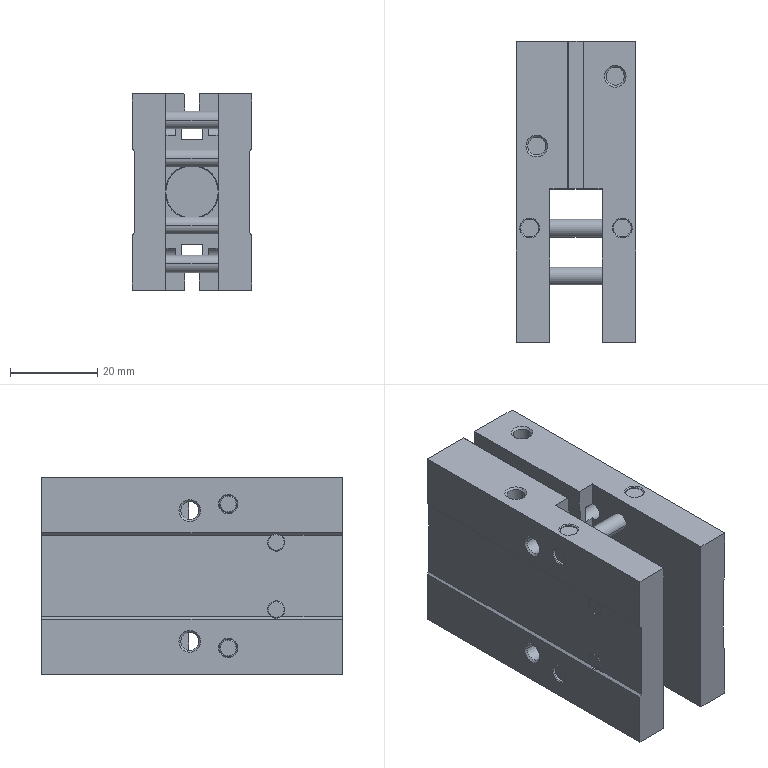Component | SolidWorks | CCDJSHFP20(NC)+(CS1-G-2)-1_CCDJSHFP20_body-1 | 1 solid | 186 faces | box 27.5 x 69 x 45 mm | volume 54359 mm3 | plane 66 | cylinder 64 | cone 56 | commonest cylinder face diameters 4 x32 4.134 x20 2 x4 21 x2 17.4 x2 20 x2 12 x2
build123d program:
from build123d import *

# Parameters (mm, degrees)
BOSS_EXTRUDE1_DEPTH     = 69
CUT_EXTRUDE1_DEPTH      = 22.5
CUT_EXTRUDE1_DEPTH_BACK = 22.5
SKETCH2_W               = 35.2
SKETCH2_H               = 12
LPATTERN1_COUNT         = 2
LPATTERN1_PITCH         = 36.715


with BuildPart() as part:
    # Sketch1 → Boss-Extrude1 (new body)
    with BuildSketch(Plane(origin=(0, 0, 0), x_dir=(0, 0, -1), z_dir=(1, 0, 0))):
        Polygon((-13.75, 9.9), (-13.25, 9.4), (-13.25, -9.4), (-13.75, -9.9), (-13.75, -22.5), (-1.9, -22.5), (-1.7, -22.3), (-1.7, -16.7), (-2.3, -16.7), (-2.3, -12), (2.3, -12), (2.3, -16.7), (1.7, -16.7), (1.7, -22.5), (13.75, -22.5), (13.75, -9.9), (13.25, -9.4), (13.25, 9.4), (13.75, 9.9), (13.75, 22.5), (1.7, 22.5), (1.7, 16.7), (2.3, 16.7), (2.3, 12), (-2.3, 12), (-2.3, 16.7), (-1.7, 16.7), (-1.7, 22.5), (-13.75, 22.5), align=None)
    extrude(amount=BOSS_EXTRUDE1_DEPTH)

    # Sketch2 → Cut-Extrude1 (cut, two sides: drawn at the far end of the back side and taken through both)
    with BuildSketch(Plane(origin=(0, 0, 0), x_dir=(1, 0, 0), z_dir=(0, 1, 0)).offset(-CUT_EXTRUDE1_DEPTH_BACK)):
        with Locations((17.6, 0)):
            Rectangle(SKETCH2_W, SKETCH2_H)
    extrude(amount=CUT_EXTRUDE1_DEPTH + CUT_EXTRUDE1_DEPTH_BACK, mode=Mode.SUBTRACT)

    # Sketch3 → Cut-Revolve1 (revolve, cut)
    with BuildSketch(Plane.XY, mode=Mode.PRIVATE) as cut_revolve1_sk:
        Polygon((35.2, 0), (35.2, 6.2), (35.4, 6), (43.9, 6), (43.9, 10), (61.2, 10), (61.2, 0), align=None)
    revolve(cut_revolve1_sk.sketch.rotate(Axis((61.2, 0, 0), (-1, 0, 0)), 270), axis=Axis((61.2, 0, 0), (-1, 0, 0)), mode=Mode.SUBTRACT)

    # Sketch4 → Cut-Revolve2 (revolve, cut)
    with BuildSketch(Plane.XY, mode=Mode.PRIVATE) as cut_revolve2_sk:
        Polygon((66.6, 0), (66.6, 8.7), (67.8, 8.7), (67.8, 10.5), (68.8, 10.5), (69, 10.7), (69, 0), align=None)
    revolve(cut_revolve2_sk.sketch.rotate(Axis((69, 0, 0), (-1, 0, 0)), 180), axis=Axis((69, 0, 0), (-1, 0, 0)), mode=Mode.SUBTRACT)

    # Sketch5 → Cut-Revolve3 (revolve, cut)
    with BuildSketch(Plane(origin=(35, 0, 0), x_dir=(0, 0, -1), z_dir=(1, 0, 0)), mode=Mode.PRIVATE) as cut_revolve3_sk:
        Polygon((-13.75, 15), (-13.75, 17.5), (-13.317, 17.067), (-3.75, 17.067), (-3.75, 15), align=None)
    revolve(cut_revolve3_sk.sketch.rotate(Axis((35, 15, 3.75), (0, 0, 1)), 270), axis=Axis((35, 15, 3.75), (0, 0, 1)), mode=Mode.SUBTRACT)

    # Sketch6 → Cut-Revolve4 (revolve, cut)
    with BuildSketch(Plane(origin=(35, 0, 0), x_dir=(0, 0, -1), z_dir=(1, 0, 0)), mode=Mode.PRIVATE) as cut_revolve4_sk:
        Polygon((3.75, 15), (3.75, 17.067), (13.317, 17.067), (13.75, 17.5), (13.75, 15), align=None)
    revolve(cut_revolve4_sk.sketch.rotate(Axis((35, 15, -13.75), (0, 0, 1)), 270), axis=Axis((35, 15, -13.75), (0, 0, 1)), mode=Mode.SUBTRACT)

    # Sketch7 → Cut-Revolve5 (revolve, cut)
    with BuildSketch(Plane(origin=(35, 0, 0), x_dir=(0, 0, -1), z_dir=(1, 0, 0)), mode=Mode.PRIVATE) as cut_revolve5_sk:
        Polygon((-13.75, -15), (-13.75, -12.5), (-13.317, -12.933), (-3.75, -12.933), (-3.75, -15), align=None)
    revolve(cut_revolve5_sk.sketch.rotate(Axis((35, -15, 3.75), (0, 0, 1)), 270), axis=Axis((35, -15, 3.75), (0, 0, 1)), mode=Mode.SUBTRACT)

    # Sketch8 → Cut-Revolve6 (revolve, cut)
    with BuildSketch(Plane(origin=(35, 0, 0), x_dir=(0, 0, -1), z_dir=(1, 0, 0)), mode=Mode.PRIVATE) as cut_revolve6_sk:
        Polygon((3.75, -15), (3.75, -12.933), (13.317, -12.933), (13.75, -12.5), (13.75, -15), align=None)
    revolve(cut_revolve6_sk.sketch.rotate(Axis((35, -15, -13.75), (0, 0, 1)), 270), axis=Axis((35, -15, -13.75), (0, 0, 1)), mode=Mode.SUBTRACT)

    # Sketch9 → Cut-Revolve7 (revolve, cut)
    with BuildSketch(Plane.XY.offset(7.5), mode=Mode.PRIVATE) as cut_revolve7_sk:
        Polygon((61.5, 9), (60.5, 9), (60.5, 12), (59.433, 12), (59.433, 22.067), (59, 22.5), (61.5, 22.5), align=None)
    revolve(cut_revolve7_sk.sketch.rotate(Axis((61.5, 22.5, 7.5), (0, -1, 0)), 90), axis=Axis((61.5, 22.5, 7.5), (0, -1, 0)), mode=Mode.SUBTRACT)

    # Sketch10 → Cut-Revolve8 (revolve, cut)
    with BuildSketch(Plane.XY.offset(-7.5), mode=Mode.PRIVATE) as cut_revolve8_sk:
        Polygon((45, 9), (44, 9), (44, 12), (42.933, 12), (42.933, 22.067), (42.5, 22.5), (45, 22.5), align=None)
    revolve(cut_revolve8_sk.sketch.rotate(Axis((45, 22.5, -7.5), (0, -1, 0)), 90), axis=Axis((45, 22.5, -7.5), (0, -1, 0)), mode=Mode.SUBTRACT)

    # Sketch11 → Cut-Revolve9 (revolve, cut)
    with BuildSketch(Plane(origin=(61, 0, 0), x_dir=(0, 0, -1), z_dir=(1, 0, 0)), mode=Mode.PRIVATE) as cut_revolve9_sk:
        Polygon((9, -22.5), (6.5, -22.5), (6.933, -22.067), (6.933, -12.5), (9, -12.5), align=None)
    revolve(cut_revolve9_sk.sketch.rotate(Axis((61, -12.5, -9), (0, -1, 0)), 180), axis=Axis((61, -12.5, -9), (0, -1, 0)), mode=Mode.SUBTRACT)

    # Sketch12 → Cut-Revolve10 (revolve, cut)
    with BuildSketch(Plane(origin=(45, 0, 0), x_dir=(0, 0, -1), z_dir=(1, 0, 0)), mode=Mode.PRIVATE) as cut_revolve10_sk:
        Polygon((-9, -22.5), (-11.5, -22.5), (-11.067, -22.067), (-11.067, -12.5), (-9, -12.5), align=None)
    revolve(cut_revolve10_sk.sketch.rotate(Axis((45, -12.5, 9), (0, -1, 0)), 180), axis=Axis((45, -12.5, 9), (0, -1, 0)), mode=Mode.SUBTRACT)

    # Sketch13 → Cut-Revolve11 (revolve, cut)
    with BuildSketch(Plane(origin=(26.2, 0, 0), x_dir=(0, 0, -1), z_dir=(1, 0, 0)), mode=Mode.PRIVATE) as cut_revolve11_sk:
        Polygon((-13.75, 16.5), (-13.75, 18.7), (-13.55, 18.5), (13.55, 18.5), (13.75, 18.7), (13.75, 16.5), align=None)
    revolve(cut_revolve11_sk.sketch.rotate(Axis((26.2, 16.5, -13.75), (0, 0, 1)), 270), axis=Axis((26.2, 16.5, -13.75), (0, 0, 1)), mode=Mode.SUBTRACT)

    # Sketch14 → Revolve1 (revolve)
    with BuildSketch(Plane(origin=(26.2, 0, 0), x_dir=(0, 0, -1), z_dir=(1, 0, 0)), mode=Mode.PRIVATE) as revolve1_sk:
        Polygon((-13.25, 16.5), (-13.25, 18.3), (-13.05, 18.5), (13.05, 18.5), (13.25, 18.3), (13.25, 16.5), align=None)
    revolve(revolve1_sk.sketch.rotate(Axis((26.2, 16.5, -13.25), (0, 0, 1)), 270), axis=Axis((26.2, 16.5, -13.25), (0, 0, 1)))

    # Sketch15 → Cut-Revolve12 (revolve, cut)
    with BuildSketch(Plane(origin=(26.2, 0, 0), x_dir=(0, 0, -1), z_dir=(1, 0, 0)), mode=Mode.PRIVATE) as cut_revolve12_sk:
        Polygon((-13.75, -16.5), (-13.75, -14.3), (-13.55, -14.5), (13.55, -14.5), (13.75, -14.3), (13.75, -16.5), align=None)
    revolve(cut_revolve12_sk.sketch.rotate(Axis((26.2, -16.5, -13.75), (0, 0, 1)), 270), axis=Axis((26.2, -16.5, -13.75), (0, 0, 1)), mode=Mode.SUBTRACT)

    # Sketch16 → Revolve2 (revolve)
    with BuildSketch(Plane(origin=(26.2, 0, 0), x_dir=(0, 0, -1), z_dir=(1, 0, 0)), mode=Mode.PRIVATE) as revolve2_sk:
        Polygon((-13.25, -16.5), (-13.25, -14.7), (-13.05, -14.5), (13.05, -14.5), (13.25, -14.7), (13.25, -16.5), align=None)
    revolve(revolve2_sk.sketch.rotate(Axis((26.2, -16.5, -13.25), (0, 0, 1)), 270), axis=Axis((26.2, -16.5, -13.25), (0, 0, 1)))

    # Sketch17 → Cut-Revolve13 (revolve, cut)
    with BuildSketch(Plane(origin=(26.2, 0, 0), x_dir=(0, 0, -1), z_dir=(1, 0, 0)), mode=Mode.PRIVATE) as cut_revolve13_sk:
        Polygon((-10.65, 22.5), (-8.4, 22.5), (-8.65, 22.25), (-8.65, 22), (-10.65, 22), align=None)
    revolve(cut_revolve13_sk.sketch.rotate(Axis((26.2, 22, 10.65), (0, 1, 0)), 180), axis=Axis((26.2, 22, 10.65), (0, 1, 0)), mode=Mode.SUBTRACT)

    # Sketch18 → Cut-Revolve14 (revolve, cut)
    with BuildSketch(Plane(origin=(26.2, 0, 0), x_dir=(0, 0, -1), z_dir=(1, 0, 0)), mode=Mode.PRIVATE) as cut_revolve14_sk:
        Polygon((10.65, 22.5), (12.9, 22.5), (12.65, 22.25), (12.65, 22), (10.65, 22), align=None)
    revolve(cut_revolve14_sk.sketch.rotate(Axis((26.2, 22, -10.65), (0, 1, 0)), 180), axis=Axis((26.2, 22, -10.65), (0, 1, 0)), mode=Mode.SUBTRACT)

    # Sketch19 → Cut-Revolve15 (revolve, cut)
    with BuildSketch(Plane(origin=(26.2, 0, 0), x_dir=(0, 0, -1), z_dir=(1, 0, 0)), mode=Mode.PRIVATE) as cut_revolve15_sk:
        Polygon((-10.65, -22), (-8.65, -22), (-8.65, -22.25), (-8.4, -22.5), (-10.65, -22.5), align=None)
    revolve(cut_revolve15_sk.sketch.rotate(Axis((26.2, -22.5, 10.65), (0, 1, 0)), 180), axis=Axis((26.2, -22.5, 10.65), (0, 1, 0)), mode=Mode.SUBTRACT)

    # Sketch20 → Cut-Revolve16 (revolve, cut)
    with BuildSketch(Plane(origin=(26.2, 0, 0), x_dir=(0, 0, -1), z_dir=(1, 0, 0)), mode=Mode.PRIVATE) as cut_revolve16_sk:
        Polygon((10.65, -22), (12.65, -22), (12.65, -22.25), (12.9, -22.5), (10.65, -22.5), align=None)
    revolve(cut_revolve16_sk.sketch.rotate(Axis((26.2, -22.5, -10.65), (0, 1, 0)), 180), axis=Axis((26.2, -22.5, -10.65), (0, 1, 0)), mode=Mode.SUBTRACT)

    # Sketch21 → Cut-Revolve17 (revolve, cut)
    with BuildSketch(Plane(origin=(15.2, 0, 0), x_dir=(0, 0, -1), z_dir=(1, 0, 0)), mode=Mode.PRIVATE) as cut_revolve17_sk:
        Polygon((-13.75, 7.7), (-13.75, 9.9), (-13.55, 9.7), (13.55, 9.7), (13.75, 9.9), (13.75, 7.7), align=None)
    revolve(cut_revolve17_sk.sketch.rotate(Axis((15.2, 7.7, -13.75), (0, 0, 1)), 270), axis=Axis((15.2, 7.7, -13.75), (0, 0, 1)), mode=Mode.SUBTRACT)

    # Sketch22 → Revolve3 (revolve)
    with BuildSketch(Plane(origin=(15.2, 0, 0), x_dir=(0, 0, -1), z_dir=(1, 0, 0)), mode=Mode.PRIVATE) as revolve3_sk:
        Polygon((-13.25, 7.7), (-13.25, 9.5), (-13.05, 9.7), (13.05, 9.7), (13.25, 9.5), (13.25, 7.7), align=None)
    revolve(revolve3_sk.sketch.rotate(Axis((15.2, 7.7, -13.25), (0, 0, 1)), 270), axis=Axis((15.2, 7.7, -13.25), (0, 0, 1)))

    # Sketch23 → Cut-Revolve18 (revolve, cut)
    with BuildSketch(Plane(origin=(15.2, 0, 0), x_dir=(0, 0, -1), z_dir=(1, 0, 0)), mode=Mode.PRIVATE) as cut_revolve18_sk:
        Polygon((-13.75, -7.7), (-13.75, -5.5), (-13.55, -5.7), (13.55, -5.7), (13.75, -5.5), (13.75, -7.7), align=None)
    revolve(cut_revolve18_sk.sketch.rotate(Axis((15.2, -7.7, -13.75), (0, 0, 1)), 270), axis=Axis((15.2, -7.7, -13.75), (0, 0, 1)), mode=Mode.SUBTRACT)

    # Sketch24 → Revolve4 (revolve)
    with BuildSketch(Plane(origin=(15.2, 0, 0), x_dir=(0, 0, -1), z_dir=(1, 0, 0)), mode=Mode.PRIVATE) as revolve4_sk:
        Polygon((-13.25, -7.7), (-13.25, -5.9), (-13.05, -5.7), (13.05, -5.7), (13.25, -5.9), (13.25, -7.7), align=None)
    revolve(revolve4_sk.sketch.rotate(Axis((15.2, -7.7, -13.25), (0, 0, 1)), 270), axis=Axis((15.2, -7.7, -13.25), (0, 0, 1)))

    # Sketch25 → Cut-Revolve19 (revolve, cut)
    with BuildSketch(Plane.XY.offset(-9), mode=Mode.PRIVATE) as cut_revolve19_sk:
        Polygon((59, 16), (59, 18.067), (68.567, 18.067), (69, 18.5), (69, 16), align=None)
    cut_revolve19 = revolve(cut_revolve19_sk.sketch.rotate(Axis((69, 16, -9), (-1, 0, 0)), 270), axis=Axis((69, 16, -9), (-1, 0, 0)), mode=Mode.SUBTRACT)

    # LPattern1: Cut-Revolve19 ×2
    with Locations(*[Vector(0, -0.8716, 0.4903) * (i * LPATTERN1_PITCH) for i in range(1, LPATTERN1_COUNT)]):
        add(cut_revolve19, mode=Mode.SUBTRACT)


solid = part.part

# Placed as in the assembly
solid = solid.moved(Location((-158.9, 291.364, -122.57), (-90, -90, 0)))